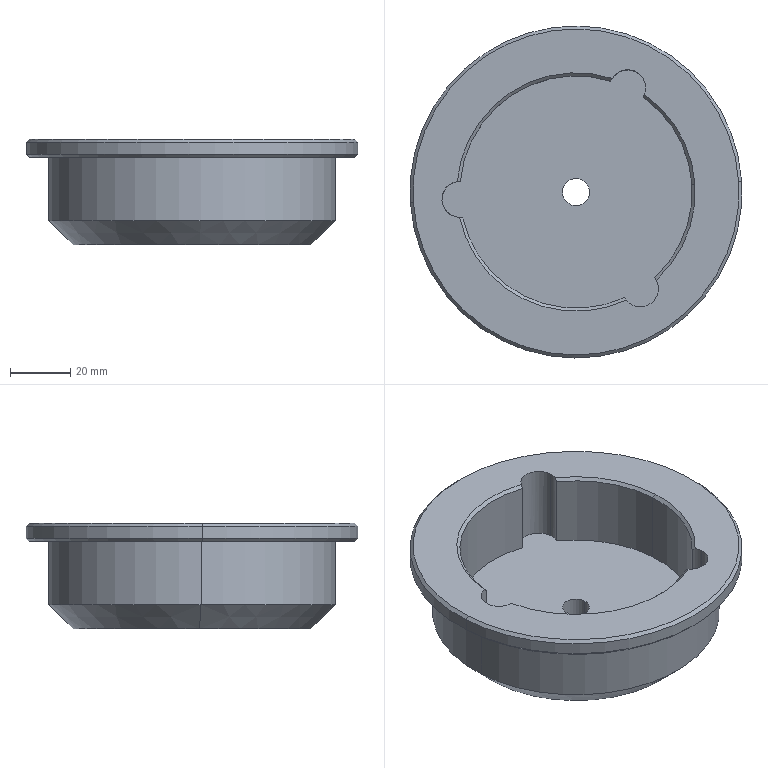Component | SolidWorks | YX-04-108GluePaperFeedingExpansionAxisCoverPlate-1 | 1 solid | 29 faces | box 110 x 110 x 35 mm | volume 131683 mm3 | cylinder 15 | cone 10 | plane 4 | commonest cylinder face diameters 12 x5 77 x4 9 x2 95 x2 110 x2 | material 45#Steel
STEP:
#1=CARTESIAN_POINT('',(-5.623,0.1486,3.819));
#2=VERTEX_POINT('',#1);
#3=CARTESIAN_POINT('',(-2.519,0.3444,3.819));
#4=VERTEX_POINT('',#3);
#5=CARTESIAN_POINT('',(-4.071,0.2465,3.819));
#6=DIRECTION('',(0.,0.,-1.));
#7=DIRECTION('',(-0.998,-0.06295,0.));
#8=AXIS2_PLACEMENT_3D('',#5,#6,#7);
#9=CIRCLE('',#8,1.555);
#10=EDGE_CURVE('',#2,#4,#9,.T.);
#11=ORIENTED_EDGE('',*,*,#10,.F.);
#12=CARTESIAN_POINT('',(-5.937,0.1288,4.134));
#13=VERTEX_POINT('',#12);
#14=CARTESIAN_POINT('',(-5.623,0.1486,3.819));
#15=DIRECTION('',(-0.7057,-0.04451,0.7071));
#16=VECTOR('',#15,39.37);
#17=LINE('',#14,#16);
#18=EDGE_CURVE('',#2,#13,#17,.T.);
#19=ORIENTED_EDGE('',*,*,#18,.T.);
#20=CARTESIAN_POINT('',(-2.204,0.3642,4.134));
#21=VERTEX_POINT('',#20);
#22=CARTESIAN_POINT('',(-4.071,0.2465,4.134));
#23=DIRECTION('',(-0.,-0.,1.));
#24=DIRECTION('',(-0.998,-0.06295,-0.));
#25=AXIS2_PLACEMENT_3D('',#22,#23,#24);
#26=CIRCLE('',#25,1.87);
#27=EDGE_CURVE('',#21,#13,#26,.T.);
#28=ORIENTED_EDGE('',*,*,#27,.F.);
#29=CARTESIAN_POINT('',(-2.519,0.3444,3.819));
#30=DIRECTION('',(0.7057,0.04451,0.7071));
#31=VECTOR('',#30,39.37);
#32=LINE('',#29,#31);
#33=EDGE_CURVE('',#4,#21,#32,.T.);
#34=ORIENTED_EDGE('',*,*,#33,.F.);
#35=EDGE_LOOP('',(#11,#19,#28,#34));
#36=FACE_OUTER_BOUND('',#35,.T.);
#37=CARTESIAN_POINT('',(-4.071,0.2465,3.819));
#38=DIRECTION('',(-0.,-0.,1.));
#39=DIRECTION('',(0.998,0.06295,0.));
#40=AXIS2_PLACEMENT_3D('',#37,#38,#39);
#41=CONICAL_SURFACE('',#40,1.555,0.7854);
#42=ADVANCED_FACE('',(#36),#41,.T.);
#43=CARTESIAN_POINT('',(-1.949,0.3804,5.197));
#44=VERTEX_POINT('',#43);
#45=CARTESIAN_POINT('',(-6.193,0.1127,5.197));
#46=VERTEX_POINT('',#45);
#47=CARTESIAN_POINT('',(-4.071,0.2465,5.197));
#48=DIRECTION('',(-0.,-0.,1.));
#49=DIRECTION('',(0.998,0.06295,0.));
#50=AXIS2_PLACEMENT_3D('',#47,#48,#49);
#51=CIRCLE('',#50,2.126);
#52=EDGE_CURVE('',#44,#46,#51,.T.);
#53=ORIENTED_EDGE('',*,*,#52,.F.);
#54=CARTESIAN_POINT('',(-1.91,0.3828,5.157));
#55=VERTEX_POINT('',#54);
#56=CARTESIAN_POINT('',(-1.949,0.3804,5.197));
#57=DIRECTION('',(0.7057,0.04451,-0.7071));
#58=VECTOR('',#57,39.37);
#59=LINE('',#56,#58);
#60=EDGE_CURVE('',#44,#55,#59,.T.);
#61=ORIENTED_EDGE('',*,*,#60,.T.);
#62=CARTESIAN_POINT('',(-6.232,0.1102,5.157));
#63=VERTEX_POINT('',#62);
#64=CARTESIAN_POINT('',(-4.071,0.2465,5.157));
#65=DIRECTION('',(0.,0.,-1.));
#66=DIRECTION('',(0.998,0.06295,0.));
#67=AXIS2_PLACEMENT_3D('',#64,#65,#66);
#68=CIRCLE('',#67,2.165);
#69=EDGE_CURVE('',#63,#55,#68,.T.);
#70=ORIENTED_EDGE('',*,*,#69,.F.);
#71=CARTESIAN_POINT('',(-6.193,0.1127,5.197));
#72=DIRECTION('',(-0.7057,-0.04451,-0.7071));
#73=VECTOR('',#72,39.37);
#74=LINE('',#71,#73);
#75=EDGE_CURVE('',#46,#63,#74,.T.);
#76=ORIENTED_EDGE('',*,*,#75,.F.);
#77=EDGE_LOOP('',(#53,#61,#70,#76));
#78=FACE_OUTER_BOUND('',#77,.T.);
#79=CARTESIAN_POINT('',(-4.071,0.2465,5.197));
#80=DIRECTION('',(0.,0.,-1.));
#81=DIRECTION('',(-0.998,-0.06295,0.));
#82=AXIS2_PLACEMENT_3D('',#79,#80,#81);
#83=CONICAL_SURFACE('',#82,2.126,0.7854);
#84=ADVANCED_FACE('',(#78),#83,.T.);
#85=CARTESIAN_POINT('',(-6.193,0.1127,4.961));
#86=VERTEX_POINT('',#85);
#87=CARTESIAN_POINT('',(-1.949,0.3804,4.961));
#88=VERTEX_POINT('',#87);
#89=CARTESIAN_POINT('',(-4.071,0.2465,4.961));
#90=DIRECTION('',(0.,0.,-1.));
#91=DIRECTION('',(-0.998,-0.06295,0.));
#92=AXIS2_PLACEMENT_3D('',#89,#90,#91);
#93=CIRCLE('',#92,2.126);
#94=EDGE_CURVE('',#86,#88,#93,.T.);
#95=ORIENTED_EDGE('',*,*,#94,.F.);
#96=CARTESIAN_POINT('',(-6.232,0.1102,5.));
#97=VERTEX_POINT('',#96);
#98=CARTESIAN_POINT('',(-6.232,0.1102,5.));
#99=DIRECTION('',(-0.7057,-0.04451,0.7071));
#100=VECTOR('',#99,39.37);
#101=LINE('',#98,#100);
#102=EDGE_CURVE('',#86,#97,#101,.T.);
#103=ORIENTED_EDGE('',*,*,#102,.T.);
#104=CARTESIAN_POINT('',(-1.91,0.3828,5.));
#105=VERTEX_POINT('',#104);
#106=CARTESIAN_POINT('',(-4.071,0.2465,5.));
#107=DIRECTION('',(-0.,-0.,1.));
#108=DIRECTION('',(-0.998,-0.06295,0.));
#109=AXIS2_PLACEMENT_3D('',#106,#107,#108);
#110=CIRCLE('',#109,2.165);
#111=EDGE_CURVE('',#105,#97,#110,.T.);
#112=ORIENTED_EDGE('',*,*,#111,.F.);
#113=CARTESIAN_POINT('',(-1.91,0.3828,5.));
#114=DIRECTION('',(0.7057,0.04451,0.7071));
#115=VECTOR('',#114,39.37);
#116=LINE('',#113,#115);
#117=EDGE_CURVE('',#88,#105,#116,.T.);
#118=ORIENTED_EDGE('',*,*,#117,.F.);
#119=EDGE_LOOP('',(#95,#103,#112,#118));
#120=FACE_OUTER_BOUND('',#119,.T.);
#121=CARTESIAN_POINT('',(-4.071,0.2465,5.));
#122=DIRECTION('',(-0.,-0.,1.));
#123=DIRECTION('',(0.998,0.06295,0.));
#124=AXIS2_PLACEMENT_3D('',#121,#122,#123);
#125=CONICAL_SURFACE('',#124,2.165,0.7854);
#126=ADVANCED_FACE('',(#120),#125,.T.);
#127=CARTESIAN_POINT('',(-2.558,0.3419,5.157));
#128=VERTEX_POINT('',#127);
#129=CARTESIAN_POINT('',(-3.194,1.483,5.157));
#130=VERTEX_POINT('',#129);
#131=CARTESIAN_POINT('',(-4.071,0.2465,5.157));
#132=DIRECTION('',(-0.,-0.,1.));
#133=DIRECTION('',(0.998,0.06295,0.));
#134=AXIS2_PLACEMENT_3D('',#131,#132,#133);
#135=CIRCLE('',#134,1.516);
#136=EDGE_CURVE('',#128,#130,#135,.T.);
#137=ORIENTED_EDGE('',*,*,#136,.F.);
#138=CARTESIAN_POINT('',(-2.519,0.3444,5.197));
#139=VERTEX_POINT('',#138);
#140=CARTESIAN_POINT('',(-2.558,0.3419,5.157));
#141=DIRECTION('',(0.7057,0.04451,0.7071));
#142=VECTOR('',#141,39.37);
#143=LINE('',#140,#142);
#144=EDGE_CURVE('',#128,#139,#143,.T.);
#145=ORIENTED_EDGE('',*,*,#144,.T.);
#146=CARTESIAN_POINT('',(-3.177,1.519,5.197));
#147=VERTEX_POINT('',#146);
#148=CARTESIAN_POINT('',(-4.071,0.2465,5.197));
#149=DIRECTION('',(0.,0.,-1.));
#150=DIRECTION('',(0.998,0.06295,0.));
#151=AXIS2_PLACEMENT_3D('',#148,#149,#150);
#152=CIRCLE('',#151,1.555);
#153=EDGE_CURVE('',#147,#139,#152,.T.);
#154=ORIENTED_EDGE('',*,*,#153,.F.);
#155=CARTESIAN_POINT('',(-3.194,1.483,5.157));
#156=CARTESIAN_POINT('',(-3.187,1.495,5.171));
#157=CARTESIAN_POINT('',(-3.182,1.506,5.184));
#158=CARTESIAN_POINT('',(-3.177,1.519,5.197));
#159=B_SPLINE_CURVE_WITH_KNOTS('',3,(#155,#156,#157,#158),.UNSPECIFIED.,.F.,.F.,(4,4),(0.,0.001423),.UNSPECIFIED.);
#160=EDGE_CURVE('',#130,#147,#159,.T.);
#161=ORIENTED_EDGE('',*,*,#160,.F.);
#162=EDGE_LOOP('',(#137,#145,#154,#161));
#163=FACE_OUTER_BOUND('',#162,.T.);
#164=CARTESIAN_POINT('',(-4.071,0.2465,5.157));
#165=DIRECTION('',(-0.,-0.,1.));
#166=DIRECTION('',(0.998,0.06295,0.));
#167=AXIS2_PLACEMENT_3D('',#164,#165,#166);
#168=CONICAL_SURFACE('',#167,1.516,0.7854);
#169=ADVANCED_FACE('',(#163),#168,.F.);
#170=CARTESIAN_POINT('',(-4.248,0.2354,4.213));
#171=VERTEX_POINT('',#170);
#172=CARTESIAN_POINT('',(-3.894,0.2577,4.213));
#173=VERTEX_POINT('',#172);
#174=CARTESIAN_POINT('',(-4.071,0.2465,4.213));
#175=DIRECTION('',(-0.,-0.,1.));
#176=DIRECTION('',(0.998,0.06295,0.));
#177=AXIS2_PLACEMENT_3D('',#174,#175,#176);
#178=CIRCLE('',#177,0.1772);
#179=EDGE_CURVE('',#171,#173,#178,.T.);
#180=ORIENTED_EDGE('',*,*,#179,.T.);
#181=CARTESIAN_POINT('',(-3.894,0.2577,3.819));
#182=VERTEX_POINT('',#181);
#183=CARTESIAN_POINT('',(-3.894,0.2577,3.819));
#184=DIRECTION('',(0.,0.,-1.));
#185=VECTOR('',#184,39.37);
#186=LINE('',#183,#185);
#187=EDGE_CURVE('',#173,#182,#186,.T.);
#188=ORIENTED_EDGE('',*,*,#187,.T.);
#189=CARTESIAN_POINT('',(-4.248,0.2354,3.819));
#190=VERTEX_POINT('',#189);
#191=CARTESIAN_POINT('',(-4.071,0.2465,3.819));
#192=DIRECTION('',(0.,0.,-1.));
#193=DIRECTION('',(-0.998,-0.06295,0.));
#194=AXIS2_PLACEMENT_3D('',#191,#192,#193);
#195=CIRCLE('',#194,0.1772);
#196=EDGE_CURVE('',#182,#190,#195,.T.);
#197=ORIENTED_EDGE('',*,*,#196,.T.);
#198=CARTESIAN_POINT('',(-4.248,0.2354,3.819));
#199=DIRECTION('',(0.,0.,-1.));
#200=VECTOR('',#199,39.37);
#201=LINE('',#198,#200);
#202=EDGE_CURVE('',#171,#190,#201,.T.);
#203=ORIENTED_EDGE('',*,*,#202,.F.);
#204=EDGE_LOOP('',(#180,#188,#197,#203));
#205=FACE_OUTER_BOUND('',#204,.T.);
#206=CARTESIAN_POINT('',(-4.071,0.2465,3.819));
#207=DIRECTION('',(0.,0.,-1.));
#208=DIRECTION('',(-0.998,-0.06295,0.));
#209=AXIS2_PLACEMENT_3D('',#206,#207,#208);
#210=CYLINDRICAL_SURFACE('',#209,0.1772);
#211=ADVANCED_FACE('',(#205),#210,.F.);
#212=CARTESIAN_POINT('',(-2.996,-1.001,4.213));
#213=VERTEX_POINT('',#212);
#214=CARTESIAN_POINT('',(-3.046,-0.8701,4.213));
#215=VERTEX_POINT('',#214);
#216=CARTESIAN_POINT('',(-3.232,-1.016,4.213));
#217=DIRECTION('',(-0.,-0.,1.));
#218=DIRECTION('',(0.998,0.06295,0.));
#219=AXIS2_PLACEMENT_3D('',#216,#217,#218);
#220=CIRCLE('',#219,0.2362);
#221=EDGE_CURVE('',#213,#215,#220,.T.);
#222=ORIENTED_EDGE('',*,*,#221,.F.);
#223=CARTESIAN_POINT('',(-2.996,-1.001,5.197));
#224=VERTEX_POINT('',#223);
#225=CARTESIAN_POINT('',(-2.996,-1.001,4.213));
#226=DIRECTION('',(-0.,-0.,1.));
#227=VECTOR('',#226,39.37);
#228=LINE('',#225,#227);
#229=EDGE_CURVE('',#213,#224,#228,.T.);
#230=ORIENTED_EDGE('',*,*,#229,.T.);
#231=CARTESIAN_POINT('',(-3.024,-0.9035,5.197));
#232=VERTEX_POINT('',#231);
#233=CARTESIAN_POINT('',(-3.232,-1.016,5.197));
#234=DIRECTION('',(-0.,-0.,1.));
#235=DIRECTION('',(0.998,0.06295,0.));
#236=AXIS2_PLACEMENT_3D('',#233,#234,#235);
#237=CIRCLE('',#236,0.2362);
#238=EDGE_CURVE('',#224,#232,#237,.T.);
#239=ORIENTED_EDGE('',*,*,#238,.T.);
#240=CARTESIAN_POINT('',(-3.046,-0.8701,5.157));
#241=VERTEX_POINT('',#240);
#242=CARTESIAN_POINT('',(-3.024,-0.9035,5.197));
#243=CARTESIAN_POINT('',(-3.03,-0.8917,5.184));
#244=CARTESIAN_POINT('',(-3.038,-0.8806,5.171));
#245=CARTESIAN_POINT('',(-3.046,-0.8701,5.157));
#246=B_SPLINE_CURVE_WITH_KNOTS('',3,(#242,#243,#244,#245),.UNSPECIFIED.,.F.,.F.,(4,4),(0.,0.001423),.UNSPECIFIED.);
#247=EDGE_CURVE('',#232,#241,#246,.T.);
#248=ORIENTED_EDGE('',*,*,#247,.T.);
#249=CARTESIAN_POINT('',(-3.046,-0.8701,4.213));
#250=DIRECTION('',(-0.,-0.,1.));
#251=VECTOR('',#250,39.37);
#252=LINE('',#249,#251);
#253=EDGE_CURVE('',#215,#241,#252,.T.);
#254=ORIENTED_EDGE('',*,*,#253,.F.);
#255=EDGE_LOOP('',(#222,#230,#239,#248,#254));
#256=FACE_OUTER_BOUND('',#255,.T.);
#257=CARTESIAN_POINT('',(-3.232,-1.016,4.213));
#258=DIRECTION('',(-0.,-0.,1.));
#259=DIRECTION('',(0.998,0.06295,0.));
#260=AXIS2_PLACEMENT_3D('',#257,#258,#259);
#261=CYLINDRICAL_SURFACE('',#260,0.2362);
#262=ADVANCED_FACE('',(#256),#261,.F.);
#263=CARTESIAN_POINT('',(-2.558,0.3419,4.213));
#264=VERTEX_POINT('',#263);
#265=CARTESIAN_POINT('',(-3.194,1.483,4.213));
#266=VERTEX_POINT('',#265);
#267=CARTESIAN_POINT('',(-4.071,0.2465,4.213));
#268=DIRECTION('',(-0.,-0.,1.));
#269=DIRECTION('',(0.998,0.06295,0.));
#270=AXIS2_PLACEMENT_3D('',#267,#268,#269);
#271=CIRCLE('',#270,1.516);
#272=EDGE_CURVE('',#264,#266,#271,.T.);
#273=ORIENTED_EDGE('',*,*,#272,.F.);
#274=CARTESIAN_POINT('',(-2.558,0.3419,4.213));
#275=DIRECTION('',(-0.,-0.,1.));
#276=VECTOR('',#275,39.37);
#277=LINE('',#274,#276);
#278=EDGE_CURVE('',#264,#128,#277,.T.);
#279=ORIENTED_EDGE('',*,*,#278,.T.);
#280=ORIENTED_EDGE('',*,*,#136,.T.);
#281=CARTESIAN_POINT('',(-3.194,1.483,4.213));
#282=DIRECTION('',(-0.,-0.,1.));
#283=VECTOR('',#282,39.37);
#284=LINE('',#281,#283);
#285=EDGE_CURVE('',#266,#130,#284,.T.);
#286=ORIENTED_EDGE('',*,*,#285,.F.);
#287=EDGE_LOOP('',(#273,#279,#280,#286));
#288=FACE_OUTER_BOUND('',#287,.T.);
#289=CARTESIAN_POINT('',(-4.071,0.2465,4.213));
#290=DIRECTION('',(-0.,-0.,1.));
#291=DIRECTION('',(0.998,0.06295,0.));
#292=AXIS2_PLACEMENT_3D('',#289,#290,#291);
#293=CYLINDRICAL_SURFACE('',#292,1.516);
#294=ADVANCED_FACE('',(#288),#293,.F.);
#295=CARTESIAN_POINT('',(-3.161,1.619,4.213));
#296=VERTEX_POINT('',#295);
#297=CARTESIAN_POINT('',(-3.616,1.693,4.213));
#298=VERTEX_POINT('',#297);
#299=CARTESIAN_POINT('',(-3.397,1.604,4.213));
#300=DIRECTION('',(-0.,-0.,1.));
#301=DIRECTION('',(0.998,0.06295,0.));
#302=AXIS2_PLACEMENT_3D('',#299,#300,#301);
#303=CIRCLE('',#302,0.2362);
#304=EDGE_CURVE('',#296,#298,#303,.T.);
#305=ORIENTED_EDGE('',*,*,#304,.F.);
#306=CARTESIAN_POINT('',(-3.161,1.619,5.197));
#307=VERTEX_POINT('',#306);
#308=CARTESIAN_POINT('',(-3.161,1.619,4.213));
#309=DIRECTION('',(-0.,-0.,1.));
#310=VECTOR('',#309,39.37);
#311=LINE('',#308,#310);
#312=EDGE_CURVE('',#296,#307,#311,.T.);
#313=ORIENTED_EDGE('',*,*,#312,.T.);
#314=CARTESIAN_POINT('',(-3.598,1.728,5.197));
#315=VERTEX_POINT('',#314);
#316=CARTESIAN_POINT('',(-3.397,1.604,5.197));
#317=DIRECTION('',(-0.,-0.,1.));
#318=DIRECTION('',(0.998,0.06295,0.));
#319=AXIS2_PLACEMENT_3D('',#316,#317,#318);
#320=CIRCLE('',#319,0.2362);
#321=EDGE_CURVE('',#307,#315,#320,.T.);
#322=ORIENTED_EDGE('',*,*,#321,.T.);
#323=CARTESIAN_POINT('',(-3.616,1.693,5.157));
#324=VERTEX_POINT('',#323);
#325=CARTESIAN_POINT('',(-3.598,1.728,5.197));
#326=CARTESIAN_POINT('',(-3.605,1.717,5.184));
#327=CARTESIAN_POINT('',(-3.611,1.705,5.171));
#328=CARTESIAN_POINT('',(-3.616,1.693,5.157));
#329=B_SPLINE_CURVE_WITH_KNOTS('',3,(#325,#326,#327,#328),.UNSPECIFIED.,.F.,.F.,(4,4),(0.,0.001423),.UNSPECIFIED.);
#330=EDGE_CURVE('',#315,#324,#329,.T.);
#331=ORIENTED_EDGE('',*,*,#330,.T.);
#332=CARTESIAN_POINT('',(-3.616,1.693,4.213));
#333=DIRECTION('',(-0.,-0.,1.));
#334=VECTOR('',#333,39.37);
#335=LINE('',#332,#334);
#336=EDGE_CURVE('',#298,#324,#335,.T.);
#337=ORIENTED_EDGE('',*,*,#336,.F.);
#338=EDGE_LOOP('',(#305,#313,#322,#331,#337));
#339=FACE_OUTER_BOUND('',#338,.T.);
#340=CARTESIAN_POINT('',(-3.397,1.604,4.213));
#341=DIRECTION('',(-0.,-0.,1.));
#342=DIRECTION('',(0.998,0.06295,0.));
#343=AXIS2_PLACEMENT_3D('',#340,#341,#342);
#344=CYLINDRICAL_SURFACE('',#343,0.2362);
#345=ADVANCED_FACE('',(#339),#344,.F.);
#346=ORIENTED_EDGE('',*,*,#27,.T.);
#347=CARTESIAN_POINT('',(-5.937,0.1288,4.961));
#348=VERTEX_POINT('',#347);
#349=CARTESIAN_POINT('',(-5.937,0.1288,3.819));
#350=DIRECTION('',(-0.,-0.,1.));
#351=VECTOR('',#350,39.37);
#352=LINE('',#349,#351);
#353=EDGE_CURVE('',#13,#348,#352,.T.);
#354=ORIENTED_EDGE('',*,*,#353,.T.);
#355=CARTESIAN_POINT('',(-2.204,0.3642,4.961));
#356=VERTEX_POINT('',#355);
#357=CARTESIAN_POINT('',(-4.071,0.2465,4.961));
#358=DIRECTION('',(0.,0.,-1.));
#359=DIRECTION('',(-0.998,-0.06295,0.));
#360=AXIS2_PLACEMENT_3D('',#357,#358,#359);
#361=CIRCLE('',#360,1.87);
#362=EDGE_CURVE('',#348,#356,#361,.T.);
#363=ORIENTED_EDGE('',*,*,#362,.T.);
#364=CARTESIAN_POINT('',(-2.204,0.3642,3.819));
#365=DIRECTION('',(-0.,-0.,1.));
#366=VECTOR('',#365,39.37);
#367=LINE('',#364,#366);
#368=EDGE_CURVE('',#21,#356,#367,.T.);
#369=ORIENTED_EDGE('',*,*,#368,.F.);
#370=EDGE_LOOP('',(#346,#354,#363,#369));
#371=FACE_OUTER_BOUND('',#370,.T.);
#372=CARTESIAN_POINT('',(-4.071,0.2465,3.819));
#373=DIRECTION('',(-0.,-0.,1.));
#374=DIRECTION('',(0.998,0.06295,0.));
#375=AXIS2_PLACEMENT_3D('',#372,#373,#374);
#376=CYLINDRICAL_SURFACE('',#375,1.87);
#377=ADVANCED_FACE('',(#371),#376,.T.);
#378=ORIENTED_EDGE('',*,*,#111,.T.);
#379=CARTESIAN_POINT('',(-6.232,0.1102,4.961));
#380=DIRECTION('',(-0.,-0.,1.));
#381=VECTOR('',#380,39.37);
#382=LINE('',#379,#381);
#383=EDGE_CURVE('',#97,#63,#382,.T.);
#384=ORIENTED_EDGE('',*,*,#383,.T.);
#385=ORIENTED_EDGE('',*,*,#69,.T.);
#386=CARTESIAN_POINT('',(-1.91,0.3828,4.961));
#387=DIRECTION('',(-0.,-0.,1.));
#388=VECTOR('',#387,39.37);
#389=LINE('',#386,#388);
#390=EDGE_CURVE('',#105,#55,#389,.T.);
#391=ORIENTED_EDGE('',*,*,#390,.F.);
#392=EDGE_LOOP('',(#378,#384,#385,#391));
#393=FACE_OUTER_BOUND('',#392,.T.);
#394=CARTESIAN_POINT('',(-4.071,0.2465,4.961));
#395=DIRECTION('',(-0.,-0.,1.));
#396=DIRECTION('',(0.998,0.06295,0.));
#397=AXIS2_PLACEMENT_3D('',#394,#395,#396);
#398=CYLINDRICAL_SURFACE('',#397,2.165);
#399=ADVANCED_FACE('',(#393),#398,.T.);
#400=ORIENTED_EDGE('',*,*,#383,.F.);
#401=CARTESIAN_POINT('',(-4.071,0.2465,5.));
#402=DIRECTION('',(-0.,-0.,1.));
#403=DIRECTION('',(-0.998,-0.06295,0.));
#404=AXIS2_PLACEMENT_3D('',#401,#402,#403);
#405=CIRCLE('',#404,2.165);
#406=EDGE_CURVE('',#97,#105,#405,.T.);
#407=ORIENTED_EDGE('',*,*,#406,.T.);
#408=ORIENTED_EDGE('',*,*,#390,.T.);
#409=CARTESIAN_POINT('',(-4.071,0.2465,5.157));
#410=DIRECTION('',(0.,0.,-1.));
#411=DIRECTION('',(0.998,0.06295,0.));
#412=AXIS2_PLACEMENT_3D('',#409,#410,#411);
#413=CIRCLE('',#412,2.165);
#414=EDGE_CURVE('',#55,#63,#413,.T.);
#415=ORIENTED_EDGE('',*,*,#414,.T.);
#416=EDGE_LOOP('',(#400,#407,#408,#415));
#417=FACE_OUTER_BOUND('',#416,.T.);
#418=CARTESIAN_POINT('',(-4.071,0.2465,4.961));
#419=DIRECTION('',(-0.,-0.,1.));
#420=DIRECTION('',(0.998,0.06295,0.));
#421=AXIS2_PLACEMENT_3D('',#418,#419,#420);
#422=CYLINDRICAL_SURFACE('',#421,2.165);
#423=ADVANCED_FACE('',(#417),#422,.T.);
#424=CARTESIAN_POINT('',(-4.071,0.2465,4.961));
#425=DIRECTION('',(0.,0.,-1.));
#426=DIRECTION('',(-0.998,-0.06295,0.));
#427=AXIS2_PLACEMENT_3D('',#424,#425,#426);
#428=CIRCLE('',#427,2.126);
#429=EDGE_CURVE('',#88,#86,#428,.T.);
#430=ORIENTED_EDGE('',*,*,#429,.T.);
#431=ORIENTED_EDGE('',*,*,#94,.T.);
#432=EDGE_LOOP('',(#430,#431));
#433=FACE_OUTER_BOUND('',#432,.T.);
#434=CARTESIAN_POINT('',(-4.071,0.2465,4.961));
#435=DIRECTION('',(0.,0.,-1.));
#436=DIRECTION('',(-0.998,-0.06295,0.));
#437=AXIS2_PLACEMENT_3D('',#434,#435,#436);
#438=CIRCLE('',#437,1.87);
#439=EDGE_CURVE('',#356,#348,#438,.T.);
#440=ORIENTED_EDGE('',*,*,#439,.F.);
#441=ORIENTED_EDGE('',*,*,#362,.F.);
#442=EDGE_LOOP('',(#440,#441));
#443=FACE_BOUND('',#442,.T.);
#444=CARTESIAN_POINT('',(-4.207,2.408,4.961));
#445=DIRECTION('',(0.,0.,-1.));
#446=DIRECTION('',(-0.998,-0.06295,-0.));
#447=AXIS2_PLACEMENT_3D('',#444,#445,#446);
#448=PLANE('',#447);
#449=ADVANCED_FACE('',(#433,#443),#448,.T.);
#450=CARTESIAN_POINT('',(-4.071,0.2465,5.197));
#451=DIRECTION('',(-0.,-0.,1.));
#452=DIRECTION('',(0.998,0.06295,0.));
#453=AXIS2_PLACEMENT_3D('',#450,#451,#452);
#454=CIRCLE('',#453,2.126);
#455=EDGE_CURVE('',#46,#44,#454,.T.);
#456=ORIENTED_EDGE('',*,*,#455,.T.);
#457=ORIENTED_EDGE('',*,*,#52,.T.);
#458=EDGE_LOOP('',(#456,#457));
#459=FACE_OUTER_BOUND('',#458,.T.);
#460=CARTESIAN_POINT('',(-3.416,-1.164,5.197));
#461=VERTEX_POINT('',#460);
#462=CARTESIAN_POINT('',(-3.232,-1.016,5.197));
#463=DIRECTION('',(-0.,-0.,1.));
#464=DIRECTION('',(0.998,0.06295,0.));
#465=AXIS2_PLACEMENT_3D('',#462,#463,#464);
#466=CIRCLE('',#465,0.2362);
#467=EDGE_CURVE('',#461,#224,#466,.T.);
#468=ORIENTED_EDGE('',*,*,#467,.F.);
#469=CARTESIAN_POINT('',(-5.59,-0.085,5.197));
#470=VERTEX_POINT('',#469);
#471=CARTESIAN_POINT('',(-4.071,0.2465,5.197));
#472=DIRECTION('',(0.,0.,-1.));
#473=DIRECTION('',(0.998,0.06295,0.));
#474=AXIS2_PLACEMENT_3D('',#471,#472,#473);
#475=CIRCLE('',#474,1.555);
#476=EDGE_CURVE('',#461,#470,#475,.T.);
#477=ORIENTED_EDGE('',*,*,#476,.T.);
#478=CARTESIAN_POINT('',(-5.62,0.3845,5.197));
#479=VERTEX_POINT('',#478);
#480=CARTESIAN_POINT('',(-5.584,0.1511,5.197));
#481=DIRECTION('',(-0.,-0.,1.));
#482=DIRECTION('',(0.998,0.06295,0.));
#483=AXIS2_PLACEMENT_3D('',#480,#481,#482);
#484=CIRCLE('',#483,0.2362);
#485=EDGE_CURVE('',#479,#470,#484,.T.);
#486=ORIENTED_EDGE('',*,*,#485,.F.);
#487=CARTESIAN_POINT('',(-4.071,0.2465,5.197));
#488=DIRECTION('',(0.,0.,-1.));
#489=DIRECTION('',(0.998,0.06295,0.));
#490=AXIS2_PLACEMENT_3D('',#487,#488,#489);
#491=CIRCLE('',#490,1.555);
#492=EDGE_CURVE('',#479,#315,#491,.T.);
#493=ORIENTED_EDGE('',*,*,#492,.T.);
#494=ORIENTED_EDGE('',*,*,#321,.F.);
#495=CARTESIAN_POINT('',(-3.397,1.604,5.197));
#496=DIRECTION('',(-0.,-0.,1.));
#497=DIRECTION('',(0.998,0.06295,0.));
#498=AXIS2_PLACEMENT_3D('',#495,#496,#497);
#499=CIRCLE('',#498,0.2362);
#500=EDGE_CURVE('',#147,#307,#499,.T.);
#501=ORIENTED_EDGE('',*,*,#500,.F.);
#502=ORIENTED_EDGE('',*,*,#153,.T.);
#503=CARTESIAN_POINT('',(-4.071,0.2465,5.197));
#504=DIRECTION('',(0.,0.,-1.));
#505=DIRECTION('',(0.998,0.06295,0.));
#506=AXIS2_PLACEMENT_3D('',#503,#504,#505);
#507=CIRCLE('',#506,1.555);
#508=EDGE_CURVE('',#139,#232,#507,.T.);
#509=ORIENTED_EDGE('',*,*,#508,.T.);
#510=ORIENTED_EDGE('',*,*,#238,.F.);
#511=EDGE_LOOP('',(#468,#477,#486,#493,#494,#501,#502,#509,#510));
#512=FACE_BOUND('',#511,.T.);
#513=CARTESIAN_POINT('',(-4.071,0.2465,5.197));
#514=DIRECTION('',(-0.,-0.,1.));
#515=DIRECTION('',(0.998,0.06295,0.));
#516=AXIS2_PLACEMENT_3D('',#513,#514,#515);
#517=PLANE('',#516);
#518=ADVANCED_FACE('',(#459,#512),#517,.T.);
#519=ORIENTED_EDGE('',*,*,#353,.F.);
#520=CARTESIAN_POINT('',(-4.071,0.2465,4.134));
#521=DIRECTION('',(-0.,-0.,1.));
#522=DIRECTION('',(-0.998,-0.06295,-0.));
#523=AXIS2_PLACEMENT_3D('',#520,#521,#522);
#524=CIRCLE('',#523,1.87);
#525=EDGE_CURVE('',#13,#21,#524,.T.);
#526=ORIENTED_EDGE('',*,*,#525,.T.);
#527=ORIENTED_EDGE('',*,*,#368,.T.);
#528=ORIENTED_EDGE('',*,*,#439,.T.);
#529=EDGE_LOOP('',(#519,#526,#527,#528));
#530=FACE_OUTER_BOUND('',#529,.T.);
#531=CARTESIAN_POINT('',(-4.071,0.2465,3.819));
#532=DIRECTION('',(-0.,-0.,1.));
#533=DIRECTION('',(0.998,0.06295,0.));
#534=AXIS2_PLACEMENT_3D('',#531,#532,#533);
#535=CYLINDRICAL_SURFACE('',#534,1.87);
#536=ADVANCED_FACE('',(#530),#535,.T.);
#537=CARTESIAN_POINT('',(-4.071,0.2465,3.819));
#538=DIRECTION('',(0.,0.,-1.));
#539=DIRECTION('',(-0.998,-0.06295,0.));
#540=AXIS2_PLACEMENT_3D('',#537,#538,#539);
#541=CIRCLE('',#540,1.555);
#542=EDGE_CURVE('',#4,#2,#541,.T.);
#543=ORIENTED_EDGE('',*,*,#542,.T.);
#544=ORIENTED_EDGE('',*,*,#10,.T.);
#545=EDGE_LOOP('',(#543,#544));
#546=FACE_OUTER_BOUND('',#545,.T.);
#547=CARTESIAN_POINT('',(-4.071,0.2465,3.819));
#548=DIRECTION('',(0.,0.,-1.));
#549=DIRECTION('',(-0.998,-0.06295,0.));
#550=AXIS2_PLACEMENT_3D('',#547,#548,#549);
#551=CIRCLE('',#550,0.1772);
#552=EDGE_CURVE('',#190,#182,#551,.T.);
#553=ORIENTED_EDGE('',*,*,#552,.F.);
#554=ORIENTED_EDGE('',*,*,#196,.F.);
#555=EDGE_LOOP('',(#553,#554));
#556=FACE_BOUND('',#555,.T.);
#557=CARTESIAN_POINT('',(-4.071,0.2465,3.819));
#558=DIRECTION('',(0.,0.,-1.));
#559=DIRECTION('',(-0.998,-0.06295,-0.));
#560=AXIS2_PLACEMENT_3D('',#557,#558,#559);
#561=PLANE('',#560);
#562=ADVANCED_FACE('',(#546,#556),#561,.T.);
#563=ORIENTED_EDGE('',*,*,#485,.T.);
#564=CARTESIAN_POINT('',(-5.55,-0.08275,5.157));
#565=VERTEX_POINT('',#564);
#566=CARTESIAN_POINT('',(-5.59,-0.085,5.197));
#567=CARTESIAN_POINT('',(-5.577,-0.08538,5.184));
#568=CARTESIAN_POINT('',(-5.563,-0.08461,5.171));
#569=CARTESIAN_POINT('',(-5.55,-0.08275,5.157));
#570=B_SPLINE_CURVE_WITH_KNOTS('',3,(#566,#567,#568,#569),.UNSPECIFIED.,.F.,.F.,(4,4),(0.,0.001423),.UNSPECIFIED.);
#571=EDGE_CURVE('',#470,#565,#570,.T.);
#572=ORIENTED_EDGE('',*,*,#571,.T.);
#573=CARTESIAN_POINT('',(-5.55,-0.08275,4.213));
#574=VERTEX_POINT('',#573);
#575=CARTESIAN_POINT('',(-5.55,-0.08275,4.213));
#576=DIRECTION('',(-0.,-0.,1.));
#577=VECTOR('',#576,39.37);
#578=LINE('',#575,#577);
#579=EDGE_CURVE('',#574,#565,#578,.T.);
#580=ORIENTED_EDGE('',*,*,#579,.F.);
#581=CARTESIAN_POINT('',(-5.58,0.3873,4.213));
#582=VERTEX_POINT('',#581);
#583=CARTESIAN_POINT('',(-5.584,0.1511,4.213));
#584=DIRECTION('',(-0.,-0.,1.));
#585=DIRECTION('',(0.998,0.06295,0.));
#586=AXIS2_PLACEMENT_3D('',#583,#584,#585);
#587=CIRCLE('',#586,0.2362);
#588=EDGE_CURVE('',#582,#574,#587,.T.);
#589=ORIENTED_EDGE('',*,*,#588,.F.);
#590=CARTESIAN_POINT('',(-5.58,0.3873,5.157));
#591=VERTEX_POINT('',#590);
#592=CARTESIAN_POINT('',(-5.58,0.3873,4.213));
#593=DIRECTION('',(-0.,-0.,1.));
#594=VECTOR('',#593,39.37);
#595=LINE('',#592,#594);
#596=EDGE_CURVE('',#582,#591,#595,.T.);
#597=ORIENTED_EDGE('',*,*,#596,.T.);
#598=CARTESIAN_POINT('',(-5.58,0.3873,5.157));
#599=CARTESIAN_POINT('',(-5.593,0.3875,5.171));
#600=CARTESIAN_POINT('',(-5.606,0.3866,5.184));
#601=CARTESIAN_POINT('',(-5.62,0.3845,5.197));
#602=B_SPLINE_CURVE_WITH_KNOTS('',3,(#598,#599,#600,#601),.UNSPECIFIED.,.F.,.F.,(4,4),(0.,0.001423),.UNSPECIFIED.);
#603=EDGE_CURVE('',#591,#479,#602,.T.);
#604=ORIENTED_EDGE('',*,*,#603,.T.);
#605=EDGE_LOOP('',(#563,#572,#580,#589,#597,#604));
#606=FACE_OUTER_BOUND('',#605,.T.);
#607=CARTESIAN_POINT('',(-5.584,0.1511,4.213));
#608=DIRECTION('',(-0.,-0.,1.));
#609=DIRECTION('',(0.998,0.06295,0.));
#610=AXIS2_PLACEMENT_3D('',#607,#608,#609);
#611=CYLINDRICAL_SURFACE('',#610,0.2362);
#612=ADVANCED_FACE('',(#606),#611,.F.);
#613=ORIENTED_EDGE('',*,*,#336,.T.);
#614=CARTESIAN_POINT('',(-4.071,0.2465,5.157));
#615=DIRECTION('',(-0.,-0.,1.));
#616=DIRECTION('',(0.998,0.06295,0.));
#617=AXIS2_PLACEMENT_3D('',#614,#615,#616);
#618=CIRCLE('',#617,1.516);
#619=EDGE_CURVE('',#324,#591,#618,.T.);
#620=ORIENTED_EDGE('',*,*,#619,.T.);
#621=ORIENTED_EDGE('',*,*,#596,.F.);
#622=CARTESIAN_POINT('',(-4.071,0.2465,4.213));
#623=DIRECTION('',(-0.,-0.,1.));
#624=DIRECTION('',(0.998,0.06295,0.));
#625=AXIS2_PLACEMENT_3D('',#622,#623,#624);
#626=CIRCLE('',#625,1.516);
#627=EDGE_CURVE('',#298,#582,#626,.T.);
#628=ORIENTED_EDGE('',*,*,#627,.F.);
#629=EDGE_LOOP('',(#613,#620,#621,#628));
#630=FACE_OUTER_BOUND('',#629,.T.);
#631=CARTESIAN_POINT('',(-4.071,0.2465,4.213));
#632=DIRECTION('',(-0.,-0.,1.));
#633=DIRECTION('',(0.998,0.06295,0.));
#634=AXIS2_PLACEMENT_3D('',#631,#632,#633);
#635=CYLINDRICAL_SURFACE('',#634,1.516);
#636=ADVANCED_FACE('',(#630),#635,.F.);
#637=ORIENTED_EDGE('',*,*,#312,.F.);
#638=CARTESIAN_POINT('',(-3.397,1.604,4.213));
#639=DIRECTION('',(-0.,-0.,1.));
#640=DIRECTION('',(0.998,0.06295,0.));
#641=AXIS2_PLACEMENT_3D('',#638,#639,#640);
#642=CIRCLE('',#641,0.2362);
#643=EDGE_CURVE('',#266,#296,#642,.T.);
#644=ORIENTED_EDGE('',*,*,#643,.F.);
#645=ORIENTED_EDGE('',*,*,#285,.T.);
#646=ORIENTED_EDGE('',*,*,#160,.T.);
#647=ORIENTED_EDGE('',*,*,#500,.T.);
#648=EDGE_LOOP('',(#637,#644,#645,#646,#647));
#649=FACE_OUTER_BOUND('',#648,.T.);
#650=CARTESIAN_POINT('',(-3.397,1.604,4.213));
#651=DIRECTION('',(-0.,-0.,1.));
#652=DIRECTION('',(0.998,0.06295,0.));
#653=AXIS2_PLACEMENT_3D('',#650,#651,#652);
#654=CYLINDRICAL_SURFACE('',#653,0.2362);
#655=ADVANCED_FACE('',(#649),#654,.F.);
#656=ORIENTED_EDGE('',*,*,#278,.F.);
#657=CARTESIAN_POINT('',(-4.071,0.2465,4.213));
#658=DIRECTION('',(-0.,-0.,1.));
#659=DIRECTION('',(0.998,0.06295,0.));
#660=AXIS2_PLACEMENT_3D('',#657,#658,#659);
#661=CIRCLE('',#660,1.516);
#662=EDGE_CURVE('',#215,#264,#661,.T.);
#663=ORIENTED_EDGE('',*,*,#662,.F.);
#664=ORIENTED_EDGE('',*,*,#253,.T.);
#665=CARTESIAN_POINT('',(-4.071,0.2465,5.157));
#666=DIRECTION('',(-0.,-0.,1.));
#667=DIRECTION('',(0.998,0.06295,0.));
#668=AXIS2_PLACEMENT_3D('',#665,#666,#667);
#669=CIRCLE('',#668,1.516);
#670=EDGE_CURVE('',#241,#128,#669,.T.);
#671=ORIENTED_EDGE('',*,*,#670,.T.);
#672=EDGE_LOOP('',(#656,#663,#664,#671));
#673=FACE_OUTER_BOUND('',#672,.T.);
#674=CARTESIAN_POINT('',(-4.071,0.2465,4.213));
#675=DIRECTION('',(-0.,-0.,1.));
#676=DIRECTION('',(0.998,0.06295,0.));
#677=AXIS2_PLACEMENT_3D('',#674,#675,#676);
#678=CYLINDRICAL_SURFACE('',#677,1.516);
#679=ADVANCED_FACE('',(#673),#678,.F.);
#680=ORIENTED_EDGE('',*,*,#229,.F.);
#681=CARTESIAN_POINT('',(-3.438,-1.131,4.213));
#682=VERTEX_POINT('',#681);
#683=CARTESIAN_POINT('',(-3.232,-1.016,4.213));
#684=DIRECTION('',(-0.,-0.,1.));
#685=DIRECTION('',(0.998,0.06295,0.));
#686=AXIS2_PLACEMENT_3D('',#683,#684,#685);
#687=CIRCLE('',#686,0.2362);
#688=EDGE_CURVE('',#682,#213,#687,.T.);
#689=ORIENTED_EDGE('',*,*,#688,.F.);
#690=CARTESIAN_POINT('',(-3.438,-1.131,5.157));
#691=VERTEX_POINT('',#690);
#692=CARTESIAN_POINT('',(-3.438,-1.131,4.213));
#693=DIRECTION('',(-0.,-0.,1.));
#694=VECTOR('',#693,39.37);
#695=LINE('',#692,#694);
#696=EDGE_CURVE('',#682,#691,#695,.T.);
#697=ORIENTED_EDGE('',*,*,#696,.T.);
#698=CARTESIAN_POINT('',(-3.438,-1.131,5.157));
#699=CARTESIAN_POINT('',(-3.432,-1.142,5.171));
#700=CARTESIAN_POINT('',(-3.424,-1.153,5.184));
#701=CARTESIAN_POINT('',(-3.416,-1.164,5.197));
#702=B_SPLINE_CURVE_WITH_KNOTS('',3,(#698,#699,#700,#701),.UNSPECIFIED.,.F.,.F.,(4,4),(0.,0.001423),.UNSPECIFIED.);
#703=EDGE_CURVE('',#691,#461,#702,.T.);
#704=ORIENTED_EDGE('',*,*,#703,.T.);
#705=ORIENTED_EDGE('',*,*,#467,.T.);
#706=EDGE_LOOP('',(#680,#689,#697,#704,#705));
#707=FACE_OUTER_BOUND('',#706,.T.);
#708=CARTESIAN_POINT('',(-3.232,-1.016,4.213));
#709=DIRECTION('',(-0.,-0.,1.));
#710=DIRECTION('',(0.998,0.06295,0.));
#711=AXIS2_PLACEMENT_3D('',#708,#709,#710);
#712=CYLINDRICAL_SURFACE('',#711,0.2362);
#713=ADVANCED_FACE('',(#707),#712,.F.);
#714=ORIENTED_EDGE('',*,*,#579,.T.);
#715=CARTESIAN_POINT('',(-4.071,0.2465,5.157));
#716=DIRECTION('',(-0.,-0.,1.));
#717=DIRECTION('',(0.998,0.06295,0.));
#718=AXIS2_PLACEMENT_3D('',#715,#716,#717);
#719=CIRCLE('',#718,1.516);
#720=EDGE_CURVE('',#565,#691,#719,.T.);
#721=ORIENTED_EDGE('',*,*,#720,.T.);
#722=ORIENTED_EDGE('',*,*,#696,.F.);
#723=CARTESIAN_POINT('',(-4.071,0.2465,4.213));
#724=DIRECTION('',(-0.,-0.,1.));
#725=DIRECTION('',(0.998,0.06295,0.));
#726=AXIS2_PLACEMENT_3D('',#723,#724,#725);
#727=CIRCLE('',#726,1.516);
#728=EDGE_CURVE('',#574,#682,#727,.T.);
#729=ORIENTED_EDGE('',*,*,#728,.F.);
#730=EDGE_LOOP('',(#714,#721,#722,#729));
#731=FACE_OUTER_BOUND('',#730,.T.);
#732=CARTESIAN_POINT('',(-4.071,0.2465,4.213));
#733=DIRECTION('',(-0.,-0.,1.));
#734=DIRECTION('',(0.998,0.06295,0.));
#735=AXIS2_PLACEMENT_3D('',#732,#733,#734);
#736=CYLINDRICAL_SURFACE('',#735,1.516);
#737=ADVANCED_FACE('',(#731),#736,.F.);
#738=ORIENTED_EDGE('',*,*,#179,.F.);
#739=CARTESIAN_POINT('',(-4.071,0.2465,4.213));
#740=DIRECTION('',(-0.,-0.,1.));
#741=DIRECTION('',(0.998,0.06295,0.));
#742=AXIS2_PLACEMENT_3D('',#739,#740,#741);
#743=CIRCLE('',#742,0.1772);
#744=EDGE_CURVE('',#173,#171,#743,.T.);
#745=ORIENTED_EDGE('',*,*,#744,.F.);
#746=EDGE_LOOP('',(#738,#745));
#747=FACE_BOUND('',#746,.T.);
#748=ORIENTED_EDGE('',*,*,#588,.T.);
#749=ORIENTED_EDGE('',*,*,#728,.T.);
#750=ORIENTED_EDGE('',*,*,#688,.T.);
#751=ORIENTED_EDGE('',*,*,#221,.T.);
#752=ORIENTED_EDGE('',*,*,#662,.T.);
#753=ORIENTED_EDGE('',*,*,#272,.T.);
#754=ORIENTED_EDGE('',*,*,#643,.T.);
#755=ORIENTED_EDGE('',*,*,#304,.T.);
#756=ORIENTED_EDGE('',*,*,#627,.T.);
#757=EDGE_LOOP('',(#748,#749,#750,#751,#752,#753,#754,#755,#756));
#758=FACE_OUTER_BOUND('',#757,.T.);
#759=CARTESIAN_POINT('',(-4.827,0.1988,4.213));
#760=DIRECTION('',(-0.,-0.,1.));
#761=DIRECTION('',(0.998,0.06295,0.));
#762=AXIS2_PLACEMENT_3D('',#759,#760,#761);
#763=PLANE('',#762);
#764=ADVANCED_FACE('',(#747,#758),#763,.T.);
#765=ORIENTED_EDGE('',*,*,#187,.F.);
#766=ORIENTED_EDGE('',*,*,#744,.T.);
#767=ORIENTED_EDGE('',*,*,#202,.T.);
#768=ORIENTED_EDGE('',*,*,#552,.T.);
#769=EDGE_LOOP('',(#765,#766,#767,#768));
#770=FACE_OUTER_BOUND('',#769,.T.);
#771=CARTESIAN_POINT('',(-4.071,0.2465,3.819));
#772=DIRECTION('',(0.,0.,-1.));
#773=DIRECTION('',(-0.998,-0.06295,0.));
#774=AXIS2_PLACEMENT_3D('',#771,#772,#773);
#775=CYLINDRICAL_SURFACE('',#774,0.1772);
#776=ADVANCED_FACE('',(#770),#775,.F.);
#777=ORIENTED_EDGE('',*,*,#571,.F.);
#778=ORIENTED_EDGE('',*,*,#476,.F.);
#779=ORIENTED_EDGE('',*,*,#703,.F.);
#780=ORIENTED_EDGE('',*,*,#720,.F.);
#781=EDGE_LOOP('',(#777,#778,#779,#780));
#782=FACE_OUTER_BOUND('',#781,.T.);
#783=CARTESIAN_POINT('',(-4.071,0.2465,5.157));
#784=DIRECTION('',(-0.,-0.,1.));
#785=DIRECTION('',(0.998,0.06295,0.));
#786=AXIS2_PLACEMENT_3D('',#783,#784,#785);
#787=CONICAL_SURFACE('',#786,1.516,0.7854);
#788=ADVANCED_FACE('',(#782),#787,.F.);
#789=ORIENTED_EDGE('',*,*,#144,.F.);
#790=ORIENTED_EDGE('',*,*,#670,.F.);
#791=ORIENTED_EDGE('',*,*,#247,.F.);
#792=ORIENTED_EDGE('',*,*,#508,.F.);
#793=EDGE_LOOP('',(#789,#790,#791,#792));
#794=FACE_OUTER_BOUND('',#793,.T.);
#795=CARTESIAN_POINT('',(-4.071,0.2465,5.157));
#796=DIRECTION('',(-0.,-0.,1.));
#797=DIRECTION('',(0.998,0.06295,0.));
#798=AXIS2_PLACEMENT_3D('',#795,#796,#797);
#799=CONICAL_SURFACE('',#798,1.516,0.7854);
#800=ADVANCED_FACE('',(#794),#799,.F.);
#801=ORIENTED_EDGE('',*,*,#102,.F.);
#802=ORIENTED_EDGE('',*,*,#429,.F.);
#803=ORIENTED_EDGE('',*,*,#117,.T.);
#804=ORIENTED_EDGE('',*,*,#406,.F.);
#805=EDGE_LOOP('',(#801,#802,#803,#804));
#806=FACE_OUTER_BOUND('',#805,.T.);
#807=CARTESIAN_POINT('',(-4.071,0.2465,5.));
#808=DIRECTION('',(-0.,-0.,1.));
#809=DIRECTION('',(0.998,0.06295,0.));
#810=AXIS2_PLACEMENT_3D('',#807,#808,#809);
#811=CONICAL_SURFACE('',#810,2.165,0.7854);
#812=ADVANCED_FACE('',(#806),#811,.T.);
#813=ORIENTED_EDGE('',*,*,#60,.F.);
#814=ORIENTED_EDGE('',*,*,#455,.F.);
#815=ORIENTED_EDGE('',*,*,#75,.T.);
#816=ORIENTED_EDGE('',*,*,#414,.F.);
#817=EDGE_LOOP('',(#813,#814,#815,#816));
#818=FACE_OUTER_BOUND('',#817,.T.);
#819=CARTESIAN_POINT('',(-4.071,0.2465,5.197));
#820=DIRECTION('',(0.,0.,-1.));
#821=DIRECTION('',(-0.998,-0.06295,0.));
#822=AXIS2_PLACEMENT_3D('',#819,#820,#821);
#823=CONICAL_SURFACE('',#822,2.126,0.7854);
#824=ADVANCED_FACE('',(#818),#823,.T.);
#825=ORIENTED_EDGE('',*,*,#330,.F.);
#826=ORIENTED_EDGE('',*,*,#492,.F.);
#827=ORIENTED_EDGE('',*,*,#603,.F.);
#828=ORIENTED_EDGE('',*,*,#619,.F.);
#829=EDGE_LOOP('',(#825,#826,#827,#828));
#830=FACE_OUTER_BOUND('',#829,.T.);
#831=CARTESIAN_POINT('',(-4.071,0.2465,5.157));
#832=DIRECTION('',(-0.,-0.,1.));
#833=DIRECTION('',(0.998,0.06295,0.));
#834=AXIS2_PLACEMENT_3D('',#831,#832,#833);
#835=CONICAL_SURFACE('',#834,1.516,0.7854);
#836=ADVANCED_FACE('',(#830),#835,.F.);
#837=ORIENTED_EDGE('',*,*,#18,.F.);
#838=ORIENTED_EDGE('',*,*,#542,.F.);
#839=ORIENTED_EDGE('',*,*,#33,.T.);
#840=ORIENTED_EDGE('',*,*,#525,.F.);
#841=EDGE_LOOP('',(#837,#838,#839,#840));
#842=FACE_OUTER_BOUND('',#841,.T.);
#843=CARTESIAN_POINT('',(-4.071,0.2465,3.819));
#844=DIRECTION('',(-0.,-0.,1.));
#845=DIRECTION('',(0.998,0.06295,0.));
#846=AXIS2_PLACEMENT_3D('',#843,#844,#845);
#847=CONICAL_SURFACE('',#846,1.555,0.7854);
#848=ADVANCED_FACE('',(#842),#847,.T.);
#849=CLOSED_SHELL('',(#42,#84,#126,#169,#211,#262,#294,#345,#377,#399,#423,#449,#518,#536,#562,#612,#636,#655,#679,#713,#737,#764,#776,#788,#800,#812,#824,#836,#848));
#850=MANIFOLD_SOLID_BREP('',#849);
#851=CARTESIAN_POINT('',(0.,0.,0.));
#852=DIRECTION('',(0.,0.,1.));
#853=DIRECTION('',(1.,0.,0.));
#854=AXIS2_PLACEMENT_3D('',#851,#852,#853);
#855=(LENGTH_UNIT()NAMED_UNIT(*)SI_UNIT($,.METRE.));
#856=LENGTH_MEASURE_WITH_UNIT(LENGTH_MEASURE(0.0254),#855);
#857=DIMENSIONAL_EXPONENTS(1.,0.,0.,0.,0.,0.,0.);
#858=(CONVERSION_BASED_UNIT('',#856)LENGTH_UNIT()NAMED_UNIT(#857));
#859=UNCERTAINTY_MEASURE_WITH_UNIT(LENGTH_MEASURE(0.00001),#858,'','');
#860=(NAMED_UNIT(*)PLANE_ANGLE_UNIT()SI_UNIT($,.RADIAN.));
#861=(NAMED_UNIT(*)SI_UNIT($,.STERADIAN.)SOLID_ANGLE_UNIT());
#862=(GEOMETRIC_REPRESENTATION_CONTEXT(3)GLOBAL_UNCERTAINTY_ASSIGNED_CONTEXT((#859))GLOBAL_UNIT_ASSIGNED_CONTEXT((#858,#860,#861))REPRESENTATION_CONTEXT('',''));
#863=ADVANCED_BREP_SHAPE_REPRESENTATION('',(#850,#854),#862);
#864=COLOUR_RGB('',0.7922,0.8196,0.9333);
#865=FILL_AREA_STYLE_COLOUR('',#864);
#866=FILL_AREA_STYLE('',(#865));
#867=SURFACE_STYLE_FILL_AREA(#866);
#868=SURFACE_SIDE_STYLE('',(#867));
#869=SURFACE_STYLE_USAGE(.BOTH.,#868);
#870=PRESENTATION_STYLE_ASSIGNMENT((#869));
#871=STYLED_ITEM('',(#870),#850);
#872=PRESENTATION_LAYER_ASSIGNMENT('','',(#871));
#873=(LENGTH_UNIT()NAMED_UNIT(*)SI_UNIT($,.METRE.));
#874=LENGTH_MEASURE_WITH_UNIT(LENGTH_MEASURE(0.0254),#873);
#875=DIMENSIONAL_EXPONENTS(1.,0.,0.,0.,0.,0.,0.);
#876=(CONVERSION_BASED_UNIT('',#874)LENGTH_UNIT()NAMED_UNIT(#875));
#877=UNCERTAINTY_MEASURE_WITH_UNIT(LENGTH_MEASURE(0.00001),#876,'','');
#878=(NAMED_UNIT(*)PLANE_ANGLE_UNIT()SI_UNIT($,.RADIAN.));
#879=(NAMED_UNIT(*)SI_UNIT($,.STERADIAN.)SOLID_ANGLE_UNIT());
#880=(GEOMETRIC_REPRESENTATION_CONTEXT(3)GLOBAL_UNCERTAINTY_ASSIGNED_CONTEXT((#877))GLOBAL_UNIT_ASSIGNED_CONTEXT((#876,#878,#879))REPRESENTATION_CONTEXT('',''));
#881=MECHANICAL_DESIGN_GEOMETRIC_PRESENTATION_REPRESENTATION('',(#871),#880);